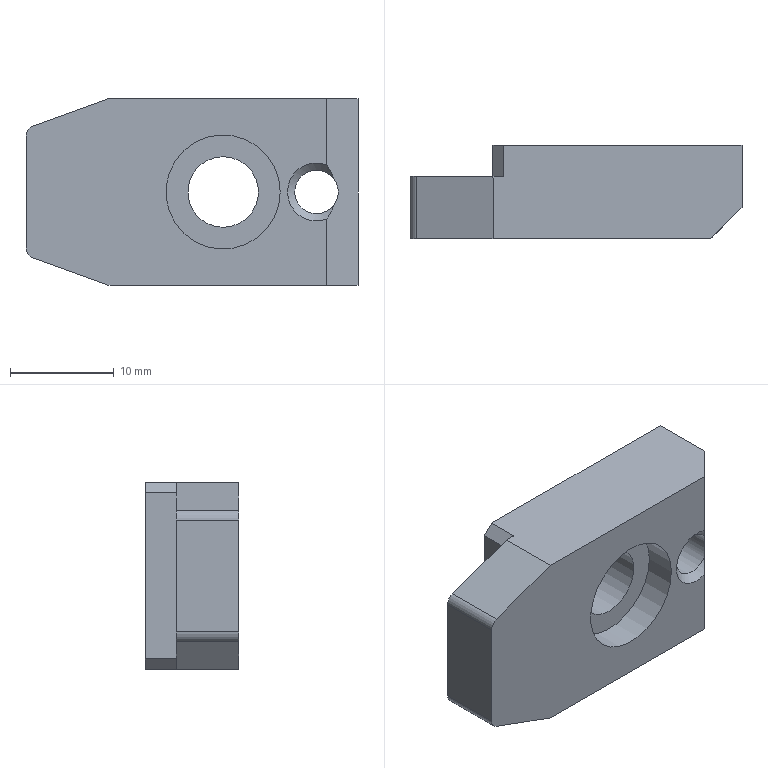CAM job | NX | mm | 3-axis | 3 set-ups | 20 operations | part box 32 x 9 x 18
set-up 1
1. Volume Based 2.5D Milling | Mill Mill5 E50R0.8 | VOLUME_BASED_2.5D_MILLING_1 | path 166 mm | 0.4078 min
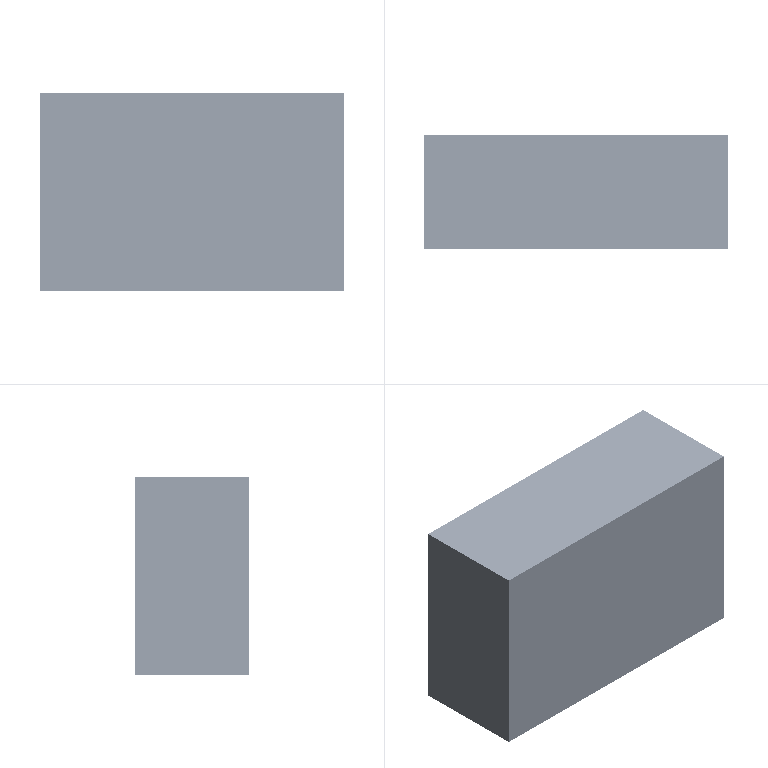2. Drilling | Mill MillChamfer DXZ-D6A90 | DRILLING_2 | path 42 mm | 0.07047 min
3. Drilling | Mill MillChamfer DXZ-D6A90 | DRILLING_3 | path 42 mm | 0.07047 min
4. Drilling | Drill DrillStandard ZT-D4.2 | DRILLING_4 | path 148.656 mm | 0.288 min
5. Drilling | Drill DrillStandard ZT-D6.8 | DRILLING_5 | path 120.258 mm | 0.3299 min
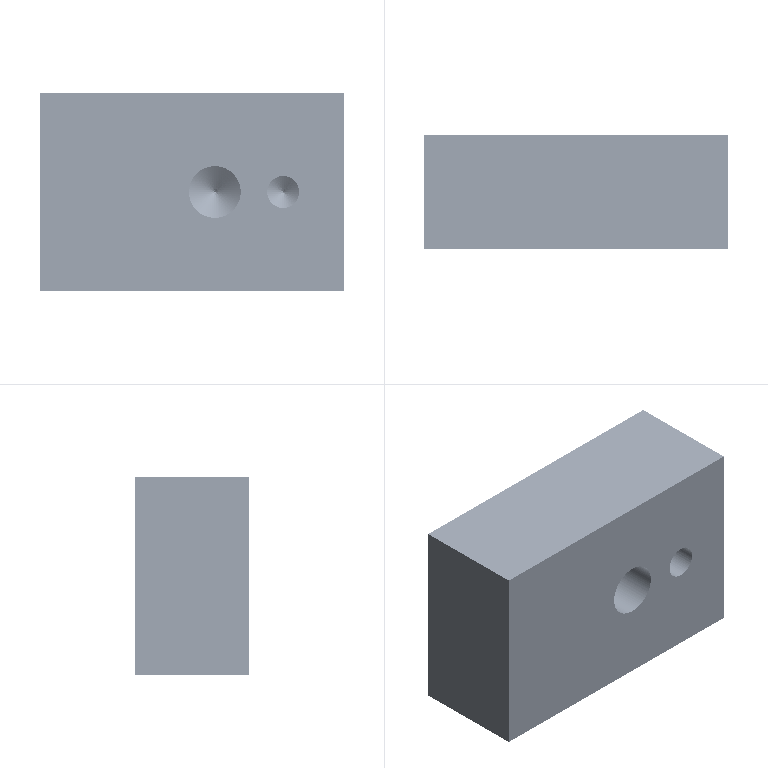6. Planar Roughing | Mill Mill5 LX-D12 | PLANAR_ROUGHING_6 | path 4002.03 mm | 1.871 min
7. Cylinder Milling | Mill Mill5 LX-D8 | CYLINDER_MILLING_7 | path 273.24 mm | 0.296 min
8. Cylinder Milling | Mill Mill5 LX-D8J | CYLINDER_MILLING_8 | path 70.252 mm | 0.08063 min
9. Planar Milling | Mill Mill5 LX-D12J | PLANAR_MILLING_9 | path 194.516 mm | 0.1801 min
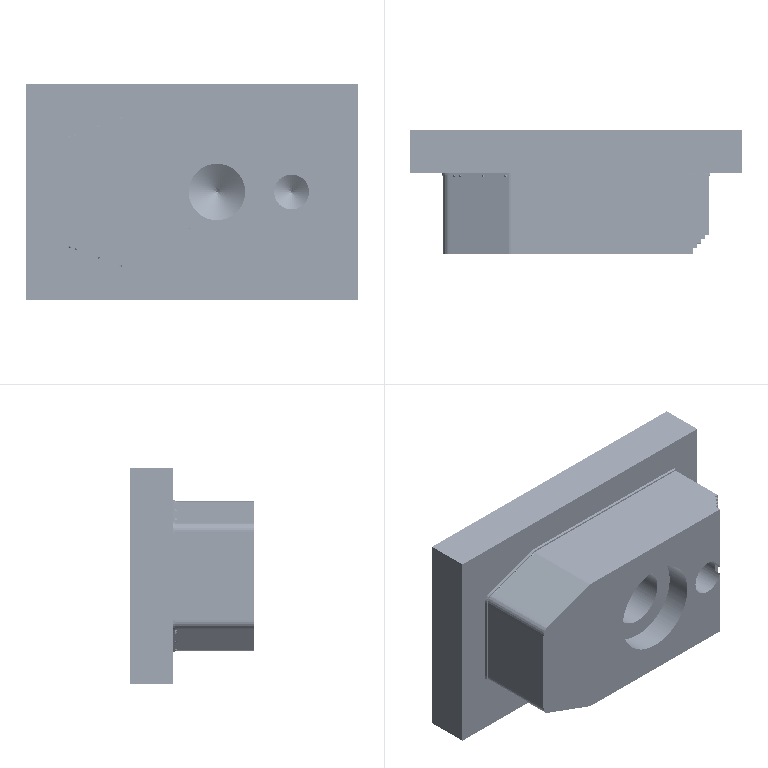10. Z-Level Milling | Mill Mill5 YB-D8R1 | Z-LEVEL_MILLING_10 | path 795.355 mm | 0.4238 min
11. Drilling | Mill MillChamfer DXZ-D10A90 | DRILLING_11 | path 45.6 mm | 0.06047 min
12. Fixed-axis Surface Contouring | Mill MillChamfer DJ-D10A90 | FIXED-AXIS_SURFACE_CONTOURING_12 | path 171.296 mm | 0.1472 min
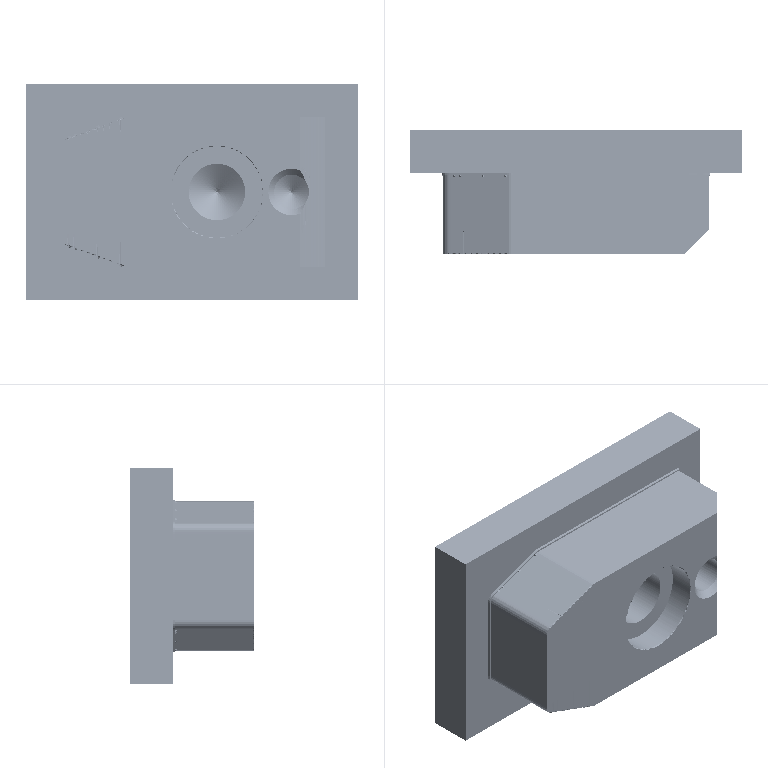13. Thread Milling | Drill DrillThreadMill M5X0.8-D4 | THREAD_MILLING_13 | path 198.738 mm | 0.2467 min
14. Thread Milling | Drill DrillThreadMill M5X0.8-D4 | THREAD_MILLING_14 | path 90.345 mm | 0.08721 min
set-up 2
15. Planar Roughing | Mill Mill5 LX-D12 | PLANAR_ROUGHING_15 | path 7046.466 mm | 3.453 min
16. Face Milling | Mill Mill5 LX-D12J | FACE_MILLING_16 | path 252 mm | 0.3573 min
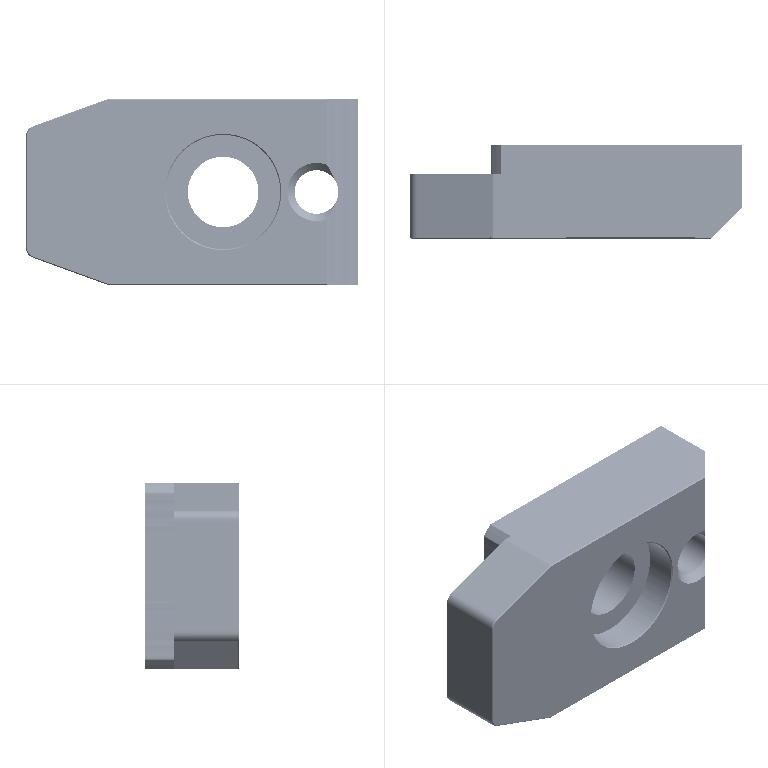17. Volume Based 2.5D Milling | Mill Mill5 LX-D12J | VOLUME_BASED_2.5D_MILLING_17 | path 100.533 mm | 0.07505 min
18. Drilling | Mill MillChamfer DXZ-D10A90 | DRILLING_18 | path 57.6 mm | 0.06167 min
19. Fixed-axis Surface Contouring | Mill MillChamfer DJ-D3A90 | FIXED-AXIS_SURFACE_CONTOURING_19 | path 295.41 mm | 0.2022 min
set-up 3
20. Planar Text | Mill Mill5 KZ-D0.5R0.25 | PLANAR_TEXT_20 | path 8932.741 mm | 2.589 min